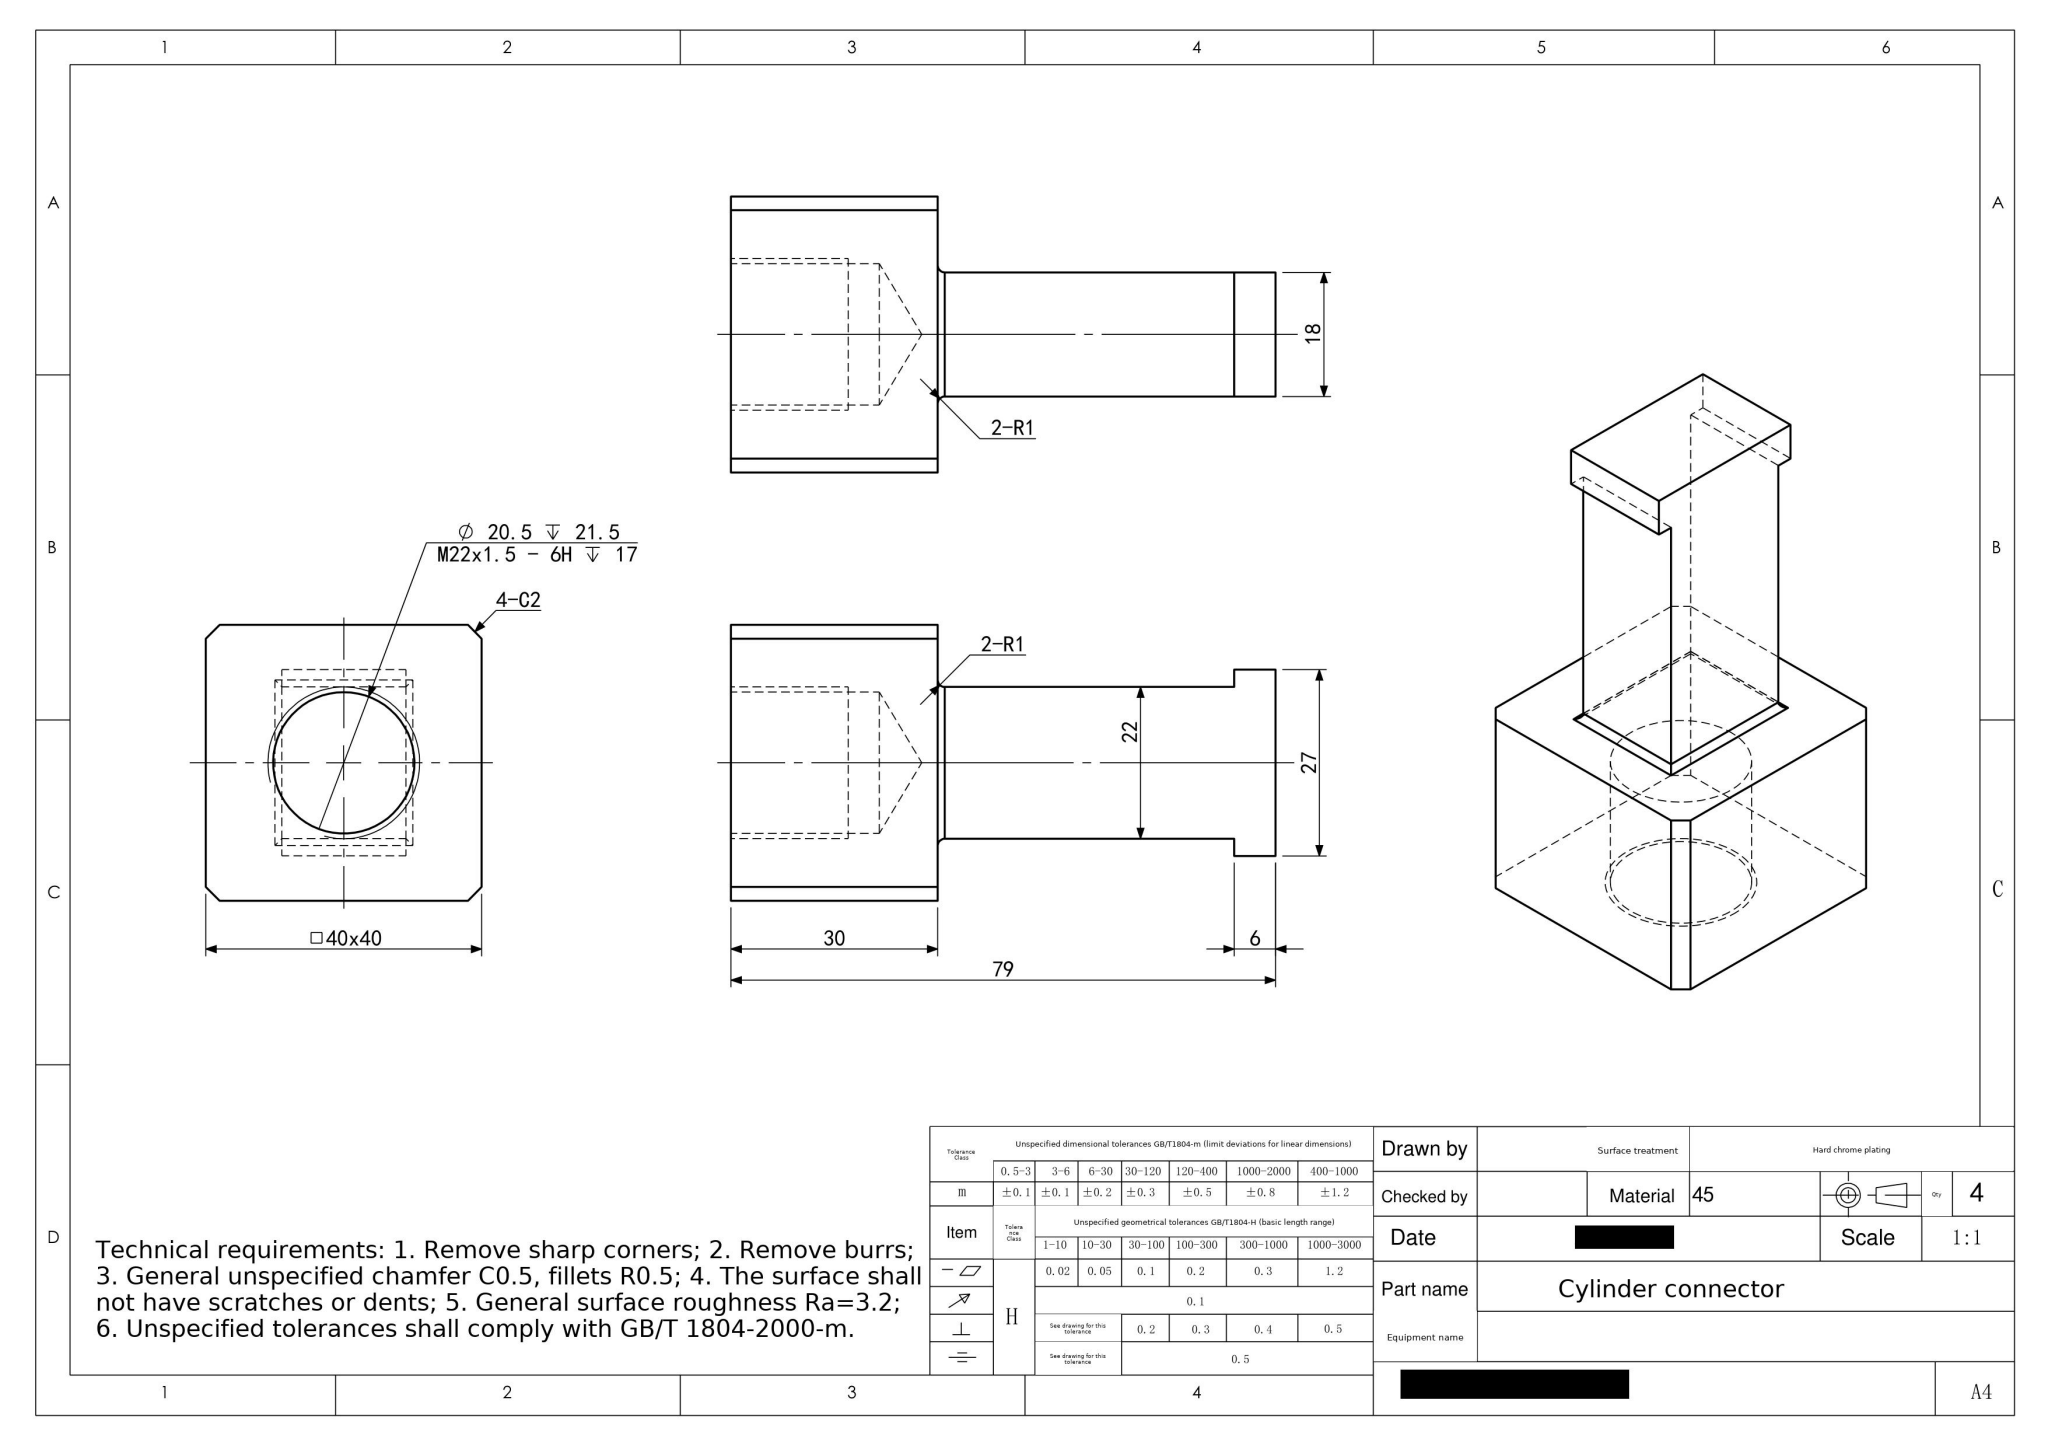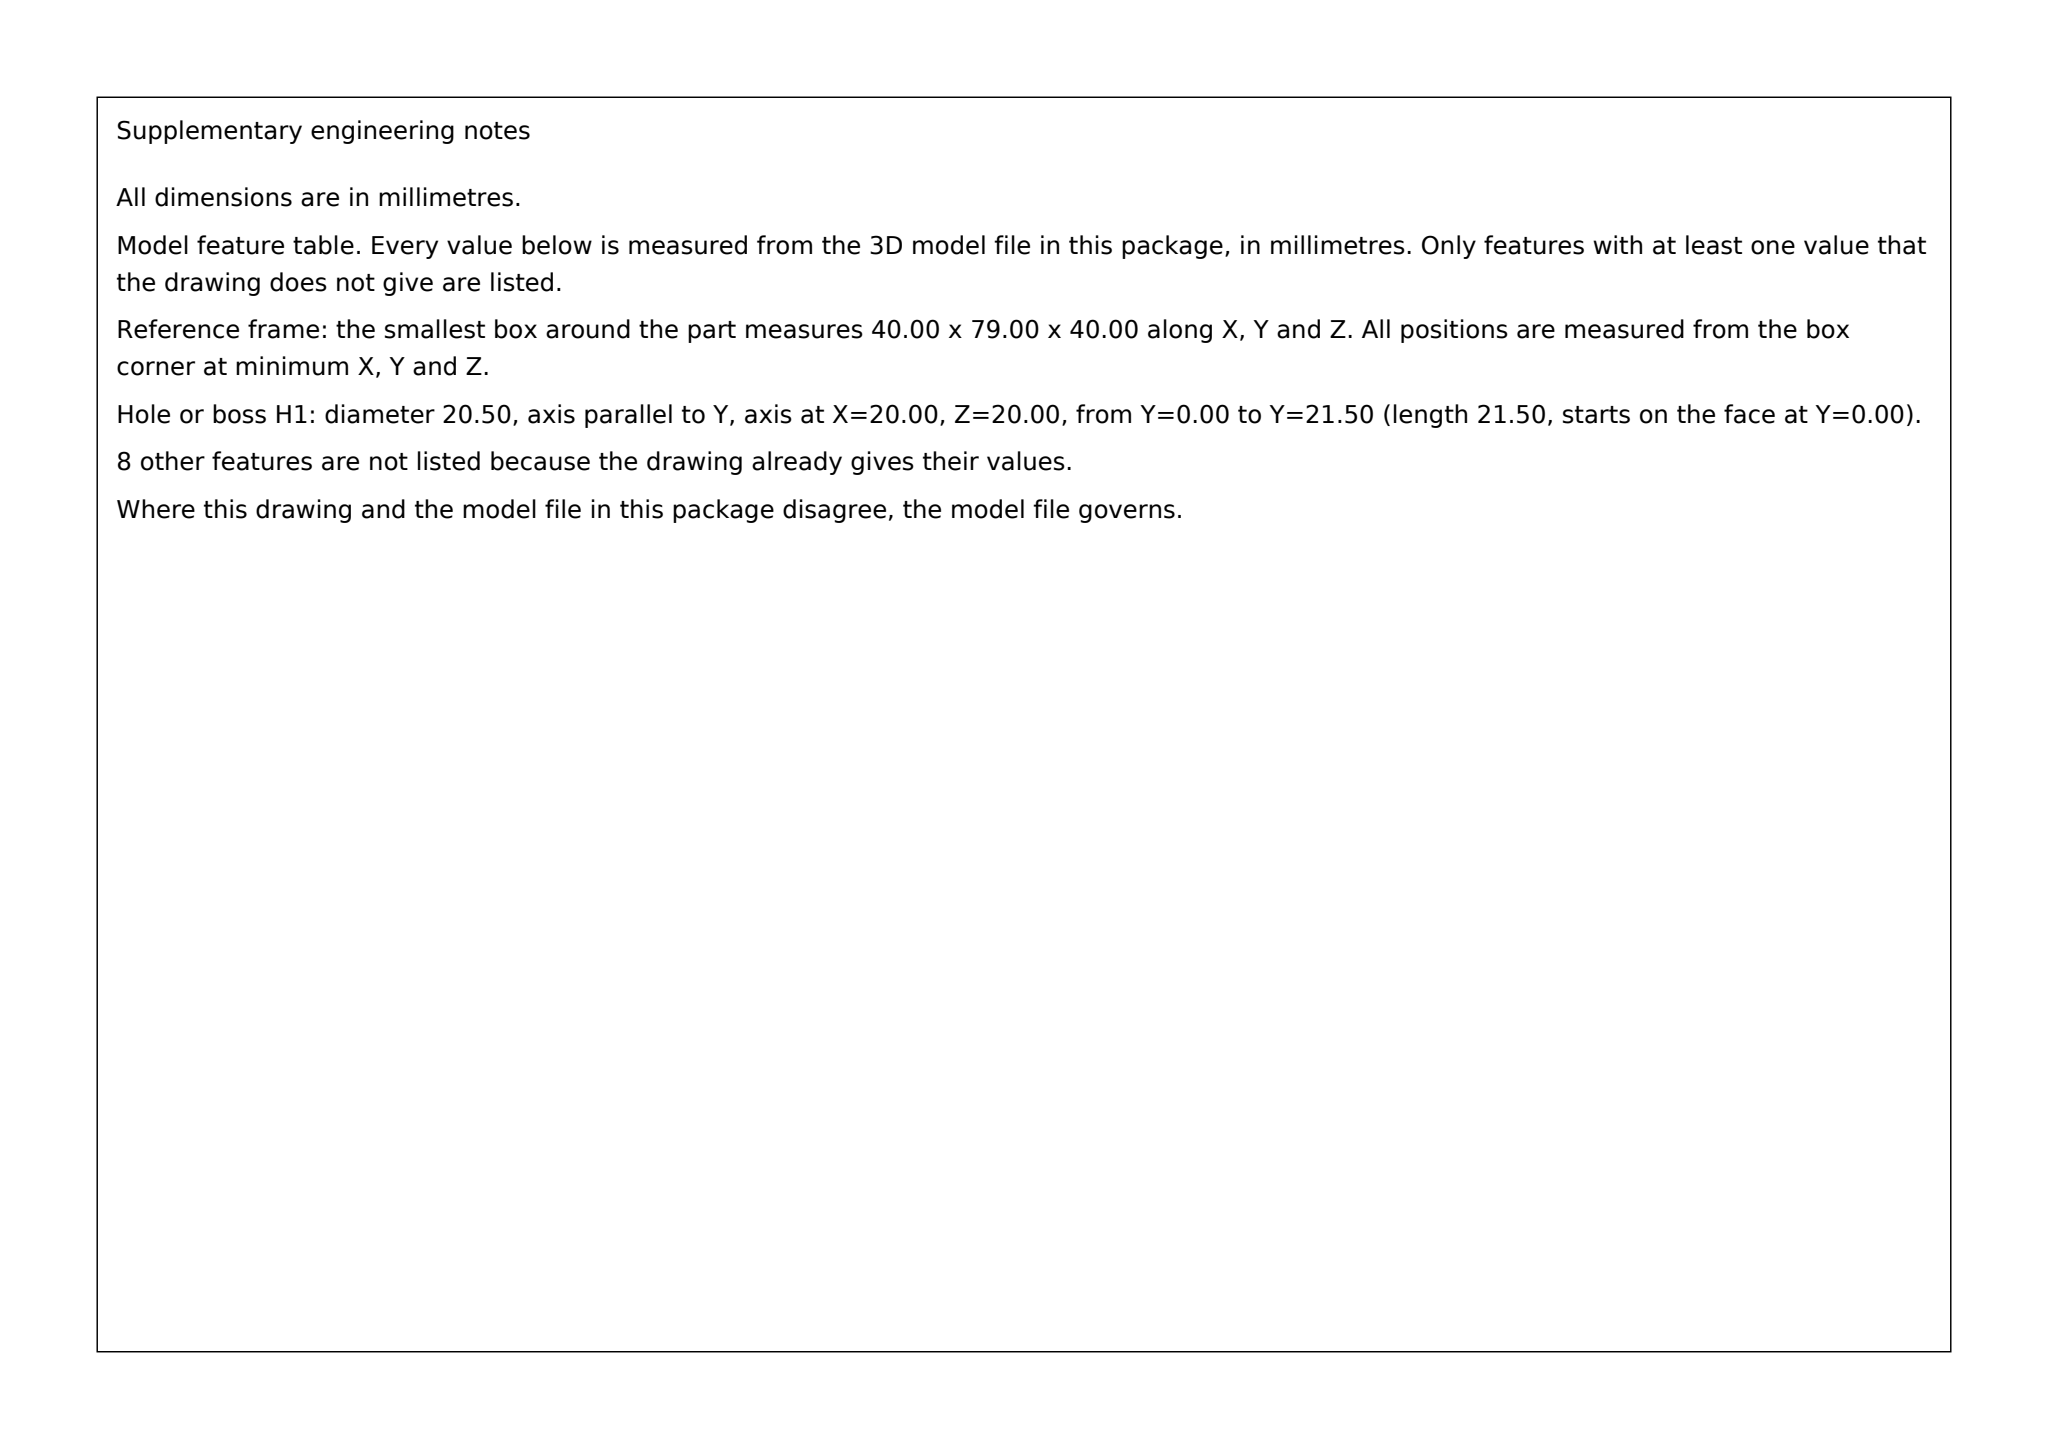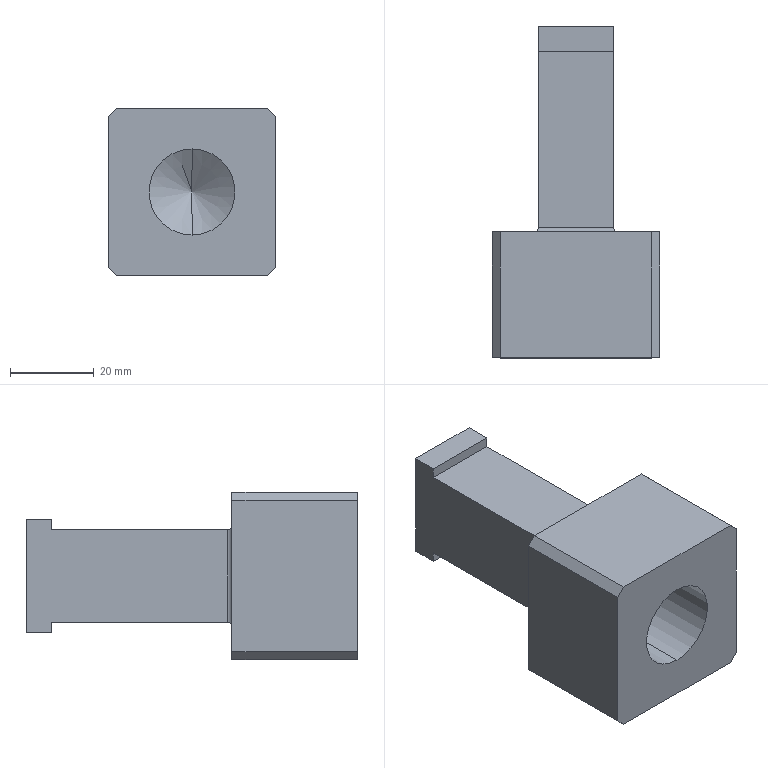Part | SolidWorks | mm | material 45 | 1 solid | 27 faces | box 40 x 79 x 40 mm | volume 59948 mm3 | plane 19 | cylinder 6 | cone 2 | commonest cylinder face diameters 2 x4 20.5 x2
build123d program:
from build123d import *

# Parameters (mm, degrees)
BOSS_EXTRUDE1_DEPTH        = 20
M22X1_5_TAPPED_HOLE1_D     = 20.5
M22X1_5_TAPPED_HOLE1_DEPTH = 21.5
M22X1_5_TAPPED_HOLE1_TIP   = 6.159
CUT_EXTRUDE1_REACH         = 85.911
SKETCH4_W                  = 11
SKETCH4_H                  = 27
FILLET1_R                  = 1
CHAMFER1_SIZE              = 2


with BuildPart() as part:
    # Sketch1 → Boss-Extrude1 (new, symmetric)
    with BuildSketch(Plane(origin=(0, 0, 0), x_dir=(0, 0, -1), z_dir=(1, 0, 0))):
        Polygon((13.5, 0), (13.5, -6), (11, -6), (11, -49), (20, -49), (20, -79), (-20, -79), (-20, -49), (-11, -49), (-11, -6), (-13.5, -6), (-13.5, 0), align=None)
    extrude(amount=BOSS_EXTRUDE1_DEPTH, both=True)

    # M22x1.5 Tapped Hole1
    with Locations(Plane(origin=(0, -79, 0), x_dir=(-1, 0, 0), z_dir=(0, -1, 0))):
        with Locations((0, 0)):
            Hole(M22X1_5_TAPPED_HOLE1_D / 2, depth=M22X1_5_TAPPED_HOLE1_DEPTH)
            with Locations((0, 0, -(M22X1_5_TAPPED_HOLE1_DEPTH + M22X1_5_TAPPED_HOLE1_TIP / 2))):  # 118° drill point
                Cone(0, M22X1_5_TAPPED_HOLE1_D / 2, M22X1_5_TAPPED_HOLE1_TIP, mode=Mode.SUBTRACT)

    # Cut-Extrude1: up to this face of the body (flat: up to its plane)
    cut_extrude1_end = Plane(part.part.faces().sort_by_distance((0, -49, -15.5))[0])
    # Sketch4 → Cut-Extrude1 (cut, up to the picked face)
    with BuildSketch(Plane(origin=(0, 0, 0), x_dir=(1, 0, 0), z_dir=(0, 1, 0)), mode=Mode.PRIVATE) as cut_extrude1_sk1:
        with Locations((-14.5, 0)):
            Rectangle(SKETCH4_W, SKETCH4_H)
    cut_extrude1_tool1 = split(extrude(cut_extrude1_sk1.sketch, amount=-CUT_EXTRUDE1_REACH, mode=Mode.PRIVATE), bisect_by=cut_extrude1_end, keep=Keep.BOTH, mode=Mode.PRIVATE)
    # Sketch4 → Cut-Extrude1 (cut, up to the picked face)
    with BuildSketch(Plane(origin=(0, 0, 0), x_dir=(1, 0, 0), z_dir=(0, 1, 0)), mode=Mode.PRIVATE) as cut_extrude1_sk2:
        with Locations((14.5, 0)):
            Rectangle(SKETCH4_W, SKETCH4_H)
    cut_extrude1_tool2 = split(extrude(cut_extrude1_sk2.sketch, amount=-CUT_EXTRUDE1_REACH, mode=Mode.PRIVATE), bisect_by=cut_extrude1_end, keep=Keep.BOTH, mode=Mode.PRIVATE)
    add(cut_extrude1_tool1.solids().sort_by(Axis((-14.5, 0, 0), (0, -1, 0)))[0], mode=Mode.SUBTRACT)
    add(cut_extrude1_tool2.solids().sort_by(Axis((14.5, 0, 0), (0, -1, 0)))[0], mode=Mode.SUBTRACT)

    # Fillet1
    fillet1_edges = [part.edges().sort_by_distance(p)[0] for p in [
        (0, -49, -11),
        (0, -49, 11),
        (-9, -49, 0),
        (9, -49, 0),
    ]]
    fillet(fillet1_edges, radius=FILLET1_R)

    # Chamfer1
    chamfer1_edges = [part.edges().sort_by_distance(p)[0] for p in [
        (-20, -64, -20),
        (-20, -64, 20),
        (20, -64, 20),
        (20, -64, -20),
    ]]
    chamfer(chamfer1_edges, length=CHAMFER1_SIZE)


solid = part.part
STEP:
#1=CARTESIAN_POINT('',(0.,-57.5,10.25));
#2=VERTEX_POINT('',#1);
#3=CARTESIAN_POINT('',(0.,-57.5,-10.25));
#4=VERTEX_POINT('',#3);
#5=CARTESIAN_POINT('',(0.,-57.5,0.));
#6=DIRECTION('',(0.,-1.,0.));
#7=DIRECTION('',(0.,0.,-1.));
#8=AXIS2_PLACEMENT_3D('',#5,#6,#7);
#9=CIRCLE('',#8,10.25);
#10=EDGE_CURVE('',#2,#4,#9,.T.);
#11=ORIENTED_EDGE('',*,*,#10,.F.);
#12=CARTESIAN_POINT('',(0.,-79.,10.25));
#13=VERTEX_POINT('',#12);
#14=CARTESIAN_POINT('',(0.,-79.,10.25));
#15=DIRECTION('',(0.,-1.,0.));
#16=VECTOR('',#15,1000.);
#17=LINE('',#14,#16);
#18=EDGE_CURVE('',#2,#13,#17,.T.);
#19=ORIENTED_EDGE('',*,*,#18,.T.);
#20=CARTESIAN_POINT('',(0.,-79.,-10.25));
#21=VERTEX_POINT('',#20);
#22=CARTESIAN_POINT('',(0.,-79.,0.));
#23=DIRECTION('',(0.,-1.,0.));
#24=DIRECTION('',(0.,0.,-1.));
#25=AXIS2_PLACEMENT_3D('',#22,#23,#24);
#26=CIRCLE('',#25,10.25);
#27=EDGE_CURVE('',#13,#21,#26,.T.);
#28=ORIENTED_EDGE('',*,*,#27,.T.);
#29=CARTESIAN_POINT('',(0.,-79.,-10.25));
#30=DIRECTION('',(0.,-1.,0.));
#31=VECTOR('',#30,1000.);
#32=LINE('',#29,#31);
#33=EDGE_CURVE('',#4,#21,#32,.T.);
#34=ORIENTED_EDGE('',*,*,#33,.F.);
#35=EDGE_LOOP('',(#11,#19,#28,#34));
#36=FACE_OUTER_BOUND('',#35,.T.);
#37=CARTESIAN_POINT('',(0.,-79.,0.));
#38=DIRECTION('',(0.,-1.,0.));
#39=DIRECTION('',(0.,0.,-1.));
#40=AXIS2_PLACEMENT_3D('',#37,#38,#39);
#41=CYLINDRICAL_SURFACE('',#40,10.25);
#42=ADVANCED_FACE('',(#36),#41,.F.);
#43=CARTESIAN_POINT('',(-0.,-51.341,0.));
#44=VERTEX_POINT('',#43);
#45=CARTESIAN_POINT('',(0.,-57.5,-10.25));
#46=DIRECTION('',(0.,-0.515,-0.8572));
#47=VECTOR('',#46,1000.);
#48=LINE('',#45,#47);
#49=EDGE_CURVE('',#44,#4,#48,.T.);
#50=ORIENTED_EDGE('',*,*,#49,.F.);
#51=CARTESIAN_POINT('',(0.,-57.5,10.25));
#52=DIRECTION('',(0.,-0.515,0.8572));
#53=VECTOR('',#52,1000.);
#54=LINE('',#51,#53);
#55=EDGE_CURVE('',#44,#2,#54,.T.);
#56=ORIENTED_EDGE('',*,*,#55,.T.);
#57=ORIENTED_EDGE('',*,*,#10,.T.);
#58=EDGE_LOOP('',(#50,#56,#57));
#59=FACE_OUTER_BOUND('',#58,.T.);
#60=CARTESIAN_POINT('',(0.,-57.5,0.));
#61=DIRECTION('',(0.,-1.,0.));
#62=DIRECTION('',(0.,0.,-1.));
#63=AXIS2_PLACEMENT_3D('',#60,#61,#62);
#64=CONICAL_SURFACE('',#63,10.25,1.03);
#65=ADVANCED_FACE('',(#59),#64,.F.);
#66=CARTESIAN_POINT('',(9.,-6.,-11.));
#67=VERTEX_POINT('',#66);
#68=CARTESIAN_POINT('',(-9.,-6.,-11.));
#69=VERTEX_POINT('',#68);
#70=CARTESIAN_POINT('',(20.,-6.,-11.));
#71=DIRECTION('',(-1.,0.,0.));
#72=VECTOR('',#71,1000.);
#73=LINE('',#70,#72);
#74=EDGE_CURVE('',#67,#69,#73,.T.);
#75=ORIENTED_EDGE('',*,*,#74,.T.);
#76=CARTESIAN_POINT('',(-9.,-6.,-13.5));
#77=VERTEX_POINT('',#76);
#78=CARTESIAN_POINT('',(-9.,-6.,-13.5));
#79=DIRECTION('',(-0.,0.,-1.));
#80=VECTOR('',#79,1000.);
#81=LINE('',#78,#80);
#82=EDGE_CURVE('',#69,#77,#81,.T.);
#83=ORIENTED_EDGE('',*,*,#82,.T.);
#84=CARTESIAN_POINT('',(9.,-6.,-13.5));
#85=VERTEX_POINT('',#84);
#86=CARTESIAN_POINT('',(20.,-6.,-13.5));
#87=DIRECTION('',(-1.,0.,0.));
#88=VECTOR('',#87,1000.);
#89=LINE('',#86,#88);
#90=EDGE_CURVE('',#85,#77,#89,.T.);
#91=ORIENTED_EDGE('',*,*,#90,.F.);
#92=CARTESIAN_POINT('',(9.,-6.,-13.5));
#93=DIRECTION('',(0.,-0.,1.));
#94=VECTOR('',#93,1000.);
#95=LINE('',#92,#94);
#96=EDGE_CURVE('',#85,#67,#95,.T.);
#97=ORIENTED_EDGE('',*,*,#96,.T.);
#98=EDGE_LOOP('',(#75,#83,#91,#97));
#99=FACE_OUTER_BOUND('',#98,.T.);
#100=CARTESIAN_POINT('',(20.,-6.,-13.5));
#101=DIRECTION('',(0.,1.,0.));
#102=DIRECTION('',(0.,-0.,1.));
#103=AXIS2_PLACEMENT_3D('',#100,#101,#102);
#104=PLANE('',#103);
#105=ADVANCED_FACE('',(#99),#104,.F.);
#106=ORIENTED_EDGE('',*,*,#90,.T.);
#107=CARTESIAN_POINT('',(-9.,0.,-13.5));
#108=VERTEX_POINT('',#107);
#109=CARTESIAN_POINT('',(-9.,-78.155,-13.5));
#110=DIRECTION('',(0.,1.,0.));
#111=VECTOR('',#110,1000.);
#112=LINE('',#109,#111);
#113=EDGE_CURVE('',#77,#108,#112,.T.);
#114=ORIENTED_EDGE('',*,*,#113,.T.);
#115=CARTESIAN_POINT('',(9.,0.,-13.5));
#116=VERTEX_POINT('',#115);
#117=CARTESIAN_POINT('',(20.,0.,-13.5));
#118=DIRECTION('',(-1.,0.,0.));
#119=VECTOR('',#118,1000.);
#120=LINE('',#117,#119);
#121=EDGE_CURVE('',#116,#108,#120,.T.);
#122=ORIENTED_EDGE('',*,*,#121,.F.);
#123=CARTESIAN_POINT('',(9.,-78.155,-13.5));
#124=DIRECTION('',(0.,1.,0.));
#125=VECTOR('',#124,1000.);
#126=LINE('',#123,#125);
#127=EDGE_CURVE('',#85,#116,#126,.T.);
#128=ORIENTED_EDGE('',*,*,#127,.F.);
#129=EDGE_LOOP('',(#106,#114,#122,#128));
#130=FACE_OUTER_BOUND('',#129,.T.);
#131=CARTESIAN_POINT('',(20.,0.,-13.5));
#132=DIRECTION('',(0.,0.,1.));
#133=DIRECTION('',(1.,0.,0.));
#134=AXIS2_PLACEMENT_3D('',#131,#132,#133);
#135=PLANE('',#134);
#136=ADVANCED_FACE('',(#130),#135,.F.);
#137=ORIENTED_EDGE('',*,*,#121,.T.);
#138=CARTESIAN_POINT('',(-9.,-0.,13.5));
#139=VERTEX_POINT('',#138);
#140=CARTESIAN_POINT('',(-9.,0.,-13.5));
#141=DIRECTION('',(-0.,0.,-1.));
#142=VECTOR('',#141,1000.);
#143=LINE('',#140,#142);
#144=EDGE_CURVE('',#139,#108,#143,.T.);
#145=ORIENTED_EDGE('',*,*,#144,.F.);
#146=CARTESIAN_POINT('',(9.,-0.,13.5));
#147=VERTEX_POINT('',#146);
#148=CARTESIAN_POINT('',(20.,-0.,13.5));
#149=DIRECTION('',(-1.,0.,0.));
#150=VECTOR('',#149,1000.);
#151=LINE('',#148,#150);
#152=EDGE_CURVE('',#147,#139,#151,.T.);
#153=ORIENTED_EDGE('',*,*,#152,.F.);
#154=CARTESIAN_POINT('',(9.,0.,-13.5));
#155=DIRECTION('',(0.,-0.,1.));
#156=VECTOR('',#155,1000.);
#157=LINE('',#154,#156);
#158=EDGE_CURVE('',#116,#147,#157,.T.);
#159=ORIENTED_EDGE('',*,*,#158,.F.);
#160=EDGE_LOOP('',(#137,#145,#153,#159));
#161=FACE_OUTER_BOUND('',#160,.T.);
#162=CARTESIAN_POINT('',(20.,0.,-13.5));
#163=DIRECTION('',(0.,-1.,-0.));
#164=DIRECTION('',(0.,0.,-1.));
#165=AXIS2_PLACEMENT_3D('',#162,#163,#164);
#166=PLANE('',#165);
#167=ADVANCED_FACE('',(#161),#166,.F.);
#168=ORIENTED_EDGE('',*,*,#152,.T.);
#169=CARTESIAN_POINT('',(-9.,-6.,13.5));
#170=VERTEX_POINT('',#169);
#171=CARTESIAN_POINT('',(-9.,-78.155,13.5));
#172=DIRECTION('',(0.,1.,0.));
#173=VECTOR('',#172,1000.);
#174=LINE('',#171,#173);
#175=EDGE_CURVE('',#170,#139,#174,.T.);
#176=ORIENTED_EDGE('',*,*,#175,.F.);
#177=CARTESIAN_POINT('',(9.,-6.,13.5));
#178=VERTEX_POINT('',#177);
#179=CARTESIAN_POINT('',(20.,-6.,13.5));
#180=DIRECTION('',(-1.,0.,0.));
#181=VECTOR('',#180,1000.);
#182=LINE('',#179,#181);
#183=EDGE_CURVE('',#178,#170,#182,.T.);
#184=ORIENTED_EDGE('',*,*,#183,.F.);
#185=CARTESIAN_POINT('',(9.,-78.155,13.5));
#186=DIRECTION('',(0.,1.,0.));
#187=VECTOR('',#186,1000.);
#188=LINE('',#185,#187);
#189=EDGE_CURVE('',#178,#147,#188,.T.);
#190=ORIENTED_EDGE('',*,*,#189,.T.);
#191=EDGE_LOOP('',(#168,#176,#184,#190));
#192=FACE_OUTER_BOUND('',#191,.T.);
#193=CARTESIAN_POINT('',(20.,-0.,13.5));
#194=DIRECTION('',(0.,0.,-1.));
#195=DIRECTION('',(-1.,0.,0.));
#196=AXIS2_PLACEMENT_3D('',#193,#194,#195);
#197=PLANE('',#196);
#198=ADVANCED_FACE('',(#192),#197,.F.);
#199=ORIENTED_EDGE('',*,*,#183,.T.);
#200=CARTESIAN_POINT('',(-9.,-6.,11.));
#201=VERTEX_POINT('',#200);
#202=CARTESIAN_POINT('',(-9.,-6.,13.5));
#203=DIRECTION('',(-0.,0.,-1.));
#204=VECTOR('',#203,1000.);
#205=LINE('',#202,#204);
#206=EDGE_CURVE('',#170,#201,#205,.T.);
#207=ORIENTED_EDGE('',*,*,#206,.T.);
#208=CARTESIAN_POINT('',(9.,-6.,11.));
#209=VERTEX_POINT('',#208);
#210=CARTESIAN_POINT('',(20.,-6.,11.));
#211=DIRECTION('',(-1.,0.,0.));
#212=VECTOR('',#211,1000.);
#213=LINE('',#210,#212);
#214=EDGE_CURVE('',#209,#201,#213,.T.);
#215=ORIENTED_EDGE('',*,*,#214,.F.);
#216=CARTESIAN_POINT('',(9.,-6.,13.5));
#217=DIRECTION('',(0.,0.,1.));
#218=VECTOR('',#217,1000.);
#219=LINE('',#216,#218);
#220=EDGE_CURVE('',#209,#178,#219,.T.);
#221=ORIENTED_EDGE('',*,*,#220,.T.);
#222=EDGE_LOOP('',(#199,#207,#215,#221));
#223=FACE_OUTER_BOUND('',#222,.T.);
#224=CARTESIAN_POINT('',(20.,-6.,13.5));
#225=DIRECTION('',(0.,1.,0.));
#226=DIRECTION('',(0.,0.,1.));
#227=AXIS2_PLACEMENT_3D('',#224,#225,#226);
#228=PLANE('',#227);
#229=ADVANCED_FACE('',(#223),#228,.F.);
#230=CARTESIAN_POINT('',(-9.,-48.,11.));
#231=VERTEX_POINT('',#230);
#232=CARTESIAN_POINT('',(-9.,-6.,11.));
#233=DIRECTION('',(-0.,-1.,-0.));
#234=VECTOR('',#233,1000.);
#235=LINE('',#232,#234);
#236=EDGE_CURVE('',#201,#231,#235,.T.);
#237=ORIENTED_EDGE('',*,*,#236,.T.);
#238=CARTESIAN_POINT('',(9.,-48.,11.));
#239=VERTEX_POINT('',#238);
#240=CARTESIAN_POINT('',(9.,-48.,11.));
#241=DIRECTION('',(1.,0.,0.));
#242=VECTOR('',#241,1000.);
#243=LINE('',#240,#242);
#244=EDGE_CURVE('',#231,#239,#243,.T.);
#245=ORIENTED_EDGE('',*,*,#244,.T.);
#246=CARTESIAN_POINT('',(9.,-6.,11.));
#247=DIRECTION('',(0.,1.,0.));
#248=VECTOR('',#247,1000.);
#249=LINE('',#246,#248);
#250=EDGE_CURVE('',#239,#209,#249,.T.);
#251=ORIENTED_EDGE('',*,*,#250,.T.);
#252=ORIENTED_EDGE('',*,*,#214,.T.);
#253=EDGE_LOOP('',(#237,#245,#251,#252));
#254=FACE_OUTER_BOUND('',#253,.T.);
#255=CARTESIAN_POINT('',(20.,-6.,11.));
#256=DIRECTION('',(0.,0.,-1.));
#257=DIRECTION('',(0.,1.,0.));
#258=AXIS2_PLACEMENT_3D('',#255,#256,#257);
#259=PLANE('',#258);
#260=ADVANCED_FACE('',(#254),#259,.F.);
#261=CARTESIAN_POINT('',(18.,-49.,20.));
#262=VERTEX_POINT('',#261);
#263=CARTESIAN_POINT('',(-18.,-49.,20.));
#264=VERTEX_POINT('',#263);
#265=CARTESIAN_POINT('',(20.,-49.,20.));
#266=DIRECTION('',(-1.,0.,0.));
#267=VECTOR('',#266,1000.);
#268=LINE('',#265,#267);
#269=EDGE_CURVE('',#262,#264,#268,.T.);
#270=ORIENTED_EDGE('',*,*,#269,.T.);
#271=CARTESIAN_POINT('',(-18.,-79.,20.));
#272=VERTEX_POINT('',#271);
#273=CARTESIAN_POINT('',(-18.,-49.,20.));
#274=DIRECTION('',(0.,-1.,0.));
#275=VECTOR('',#274,1000.);
#276=LINE('',#273,#275);
#277=EDGE_CURVE('',#264,#272,#276,.T.);
#278=ORIENTED_EDGE('',*,*,#277,.T.);
#279=CARTESIAN_POINT('',(18.,-79.,20.));
#280=VERTEX_POINT('',#279);
#281=CARTESIAN_POINT('',(20.,-79.,20.));
#282=DIRECTION('',(-1.,0.,0.));
#283=VECTOR('',#282,1000.);
#284=LINE('',#281,#283);
#285=EDGE_CURVE('',#280,#272,#284,.T.);
#286=ORIENTED_EDGE('',*,*,#285,.F.);
#287=CARTESIAN_POINT('',(18.,-49.,20.));
#288=DIRECTION('',(0.,1.,0.));
#289=VECTOR('',#288,1000.);
#290=LINE('',#287,#289);
#291=EDGE_CURVE('',#280,#262,#290,.T.);
#292=ORIENTED_EDGE('',*,*,#291,.T.);
#293=EDGE_LOOP('',(#270,#278,#286,#292));
#294=FACE_OUTER_BOUND('',#293,.T.);
#295=CARTESIAN_POINT('',(20.,-49.,20.));
#296=DIRECTION('',(0.,0.,-1.));
#297=DIRECTION('',(-1.,0.,0.));
#298=AXIS2_PLACEMENT_3D('',#295,#296,#297);
#299=PLANE('',#298);
#300=ADVANCED_FACE('',(#294),#299,.F.);
#301=CARTESIAN_POINT('',(0.,-79.,0.));
#302=DIRECTION('',(0.,-1.,0.));
#303=DIRECTION('',(0.,0.,-1.));
#304=AXIS2_PLACEMENT_3D('',#301,#302,#303);
#305=CIRCLE('',#304,10.25);
#306=EDGE_CURVE('',#21,#13,#305,.T.);
#307=ORIENTED_EDGE('',*,*,#306,.F.);
#308=ORIENTED_EDGE('',*,*,#27,.F.);
#309=EDGE_LOOP('',(#307,#308));
#310=FACE_BOUND('',#309,.T.);
#311=ORIENTED_EDGE('',*,*,#285,.T.);
#312=CARTESIAN_POINT('',(-20.,-79.,18.));
#313=VERTEX_POINT('',#312);
#314=CARTESIAN_POINT('',(-18.,-79.,20.));
#315=DIRECTION('',(-0.7071,0.,-0.7071));
#316=VECTOR('',#315,1000.);
#317=LINE('',#314,#316);
#318=EDGE_CURVE('',#272,#313,#317,.T.);
#319=ORIENTED_EDGE('',*,*,#318,.T.);
#320=CARTESIAN_POINT('',(-20.,-79.,-18.));
#321=VERTEX_POINT('',#320);
#322=CARTESIAN_POINT('',(-20.,-79.,20.));
#323=DIRECTION('',(0.,0.,-1.));
#324=VECTOR('',#323,1000.);
#325=LINE('',#322,#324);
#326=EDGE_CURVE('',#313,#321,#325,.T.);
#327=ORIENTED_EDGE('',*,*,#326,.T.);
#328=CARTESIAN_POINT('',(-18.,-79.,-20.));
#329=VERTEX_POINT('',#328);
#330=CARTESIAN_POINT('',(-18.,-79.,-20.));
#331=DIRECTION('',(0.7071,0.,-0.7071));
#332=VECTOR('',#331,1000.);
#333=LINE('',#330,#332);
#334=EDGE_CURVE('',#321,#329,#333,.T.);
#335=ORIENTED_EDGE('',*,*,#334,.T.);
#336=CARTESIAN_POINT('',(18.,-79.,-20.));
#337=VERTEX_POINT('',#336);
#338=CARTESIAN_POINT('',(20.,-79.,-20.));
#339=DIRECTION('',(-1.,0.,0.));
#340=VECTOR('',#339,1000.);
#341=LINE('',#338,#340);
#342=EDGE_CURVE('',#337,#329,#341,.T.);
#343=ORIENTED_EDGE('',*,*,#342,.F.);
#344=CARTESIAN_POINT('',(20.,-79.,-18.));
#345=VERTEX_POINT('',#344);
#346=CARTESIAN_POINT('',(20.,-79.,-18.));
#347=DIRECTION('',(0.7071,0.,0.7071));
#348=VECTOR('',#347,1000.);
#349=LINE('',#346,#348);
#350=EDGE_CURVE('',#337,#345,#349,.T.);
#351=ORIENTED_EDGE('',*,*,#350,.T.);
#352=CARTESIAN_POINT('',(20.,-79.,18.));
#353=VERTEX_POINT('',#352);
#354=CARTESIAN_POINT('',(20.,-79.,20.));
#355=DIRECTION('',(0.,0.,-1.));
#356=VECTOR('',#355,1000.);
#357=LINE('',#354,#356);
#358=EDGE_CURVE('',#353,#345,#357,.T.);
#359=ORIENTED_EDGE('',*,*,#358,.F.);
#360=CARTESIAN_POINT('',(20.,-79.,18.));
#361=DIRECTION('',(-0.7071,0.,0.7071));
#362=VECTOR('',#361,1000.);
#363=LINE('',#360,#362);
#364=EDGE_CURVE('',#353,#280,#363,.T.);
#365=ORIENTED_EDGE('',*,*,#364,.T.);
#366=EDGE_LOOP('',(#311,#319,#327,#335,#343,#351,#359,#365));
#367=FACE_OUTER_BOUND('',#366,.T.);
#368=CARTESIAN_POINT('',(20.,-79.,20.));
#369=DIRECTION('',(0.,1.,0.));
#370=DIRECTION('',(0.,0.,1.));
#371=AXIS2_PLACEMENT_3D('',#368,#369,#370);
#372=PLANE('',#371);
#373=ADVANCED_FACE('',(#310,#367),#372,.F.);
#374=CARTESIAN_POINT('',(18.,-49.,-20.));
#375=VERTEX_POINT('',#374);
#376=CARTESIAN_POINT('',(-18.,-49.,-20.));
#377=VERTEX_POINT('',#376);
#378=CARTESIAN_POINT('',(20.,-49.,-20.));
#379=DIRECTION('',(-1.,0.,0.));
#380=VECTOR('',#379,1000.);
#381=LINE('',#378,#380);
#382=EDGE_CURVE('',#375,#377,#381,.T.);
#383=ORIENTED_EDGE('',*,*,#382,.F.);
#384=CARTESIAN_POINT('',(18.,-79.,-20.));
#385=DIRECTION('',(0.,-1.,-0.));
#386=VECTOR('',#385,1000.);
#387=LINE('',#384,#386);
#388=EDGE_CURVE('',#375,#337,#387,.T.);
#389=ORIENTED_EDGE('',*,*,#388,.T.);
#390=ORIENTED_EDGE('',*,*,#342,.T.);
#391=CARTESIAN_POINT('',(-18.,-49.,-20.));
#392=DIRECTION('',(0.,1.,0.));
#393=VECTOR('',#392,1000.);
#394=LINE('',#391,#393);
#395=EDGE_CURVE('',#329,#377,#394,.T.);
#396=ORIENTED_EDGE('',*,*,#395,.T.);
#397=EDGE_LOOP('',(#383,#389,#390,#396));
#398=FACE_OUTER_BOUND('',#397,.T.);
#399=CARTESIAN_POINT('',(20.,-49.,-20.));
#400=DIRECTION('',(0.,-0.,1.));
#401=DIRECTION('',(0.,-1.,-0.));
#402=AXIS2_PLACEMENT_3D('',#399,#400,#401);
#403=PLANE('',#402);
#404=ADVANCED_FACE('',(#398),#403,.F.);
#405=CARTESIAN_POINT('',(10.,-49.,-12.));
#406=VERTEX_POINT('',#405);
#407=CARTESIAN_POINT('',(10.,-49.,12.));
#408=VERTEX_POINT('',#407);
#409=CARTESIAN_POINT('',(10.,-49.,11.));
#410=DIRECTION('',(0.,0.,1.));
#411=VECTOR('',#410,1000.);
#412=LINE('',#409,#411);
#413=EDGE_CURVE('',#406,#408,#412,.T.);
#414=ORIENTED_EDGE('',*,*,#413,.T.);
#415=CARTESIAN_POINT('',(-10.,-49.,12.));
#416=VERTEX_POINT('',#415);
#417=CARTESIAN_POINT('',(-9.,-49.,12.));
#418=DIRECTION('',(-1.,0.,0.));
#419=VECTOR('',#418,1000.);
#420=LINE('',#417,#419);
#421=EDGE_CURVE('',#408,#416,#420,.T.);
#422=ORIENTED_EDGE('',*,*,#421,.T.);
#423=CARTESIAN_POINT('',(-10.,-49.,-12.));
#424=VERTEX_POINT('',#423);
#425=CARTESIAN_POINT('',(-10.,-49.,-11.));
#426=DIRECTION('',(-0.,0.,-1.));
#427=VECTOR('',#426,1000.);
#428=LINE('',#425,#427);
#429=EDGE_CURVE('',#416,#424,#428,.T.);
#430=ORIENTED_EDGE('',*,*,#429,.T.);
#431=CARTESIAN_POINT('',(9.,-49.,-12.));
#432=DIRECTION('',(1.,0.,0.));
#433=VECTOR('',#432,1000.);
#434=LINE('',#431,#433);
#435=EDGE_CURVE('',#424,#406,#434,.T.);
#436=ORIENTED_EDGE('',*,*,#435,.T.);
#437=EDGE_LOOP('',(#414,#422,#430,#436));
#438=FACE_BOUND('',#437,.T.);
#439=CARTESIAN_POINT('',(-20.,-49.,-18.));
#440=VERTEX_POINT('',#439);
#441=CARTESIAN_POINT('',(-20.,-49.,18.));
#442=VERTEX_POINT('',#441);
#443=CARTESIAN_POINT('',(-20.,-49.,-11.));
#444=DIRECTION('',(0.,0.,1.));
#445=VECTOR('',#444,1000.);
#446=LINE('',#443,#445);
#447=EDGE_CURVE('',#440,#442,#446,.T.);
#448=ORIENTED_EDGE('',*,*,#447,.T.);
#449=CARTESIAN_POINT('',(-18.,-49.,20.));
#450=DIRECTION('',(0.7071,0.,0.7071));
#451=VECTOR('',#450,1000.);
#452=LINE('',#449,#451);
#453=EDGE_CURVE('',#442,#264,#452,.T.);
#454=ORIENTED_EDGE('',*,*,#453,.T.);
#455=ORIENTED_EDGE('',*,*,#269,.F.);
#456=CARTESIAN_POINT('',(20.,-49.,18.));
#457=VERTEX_POINT('',#456);
#458=CARTESIAN_POINT('',(20.,-49.,18.));
#459=DIRECTION('',(0.7071,0.,-0.7071));
#460=VECTOR('',#459,1000.);
#461=LINE('',#458,#460);
#462=EDGE_CURVE('',#262,#457,#461,.T.);
#463=ORIENTED_EDGE('',*,*,#462,.T.);
#464=CARTESIAN_POINT('',(20.,-49.,-18.));
#465=VERTEX_POINT('',#464);
#466=CARTESIAN_POINT('',(20.,-49.,11.));
#467=DIRECTION('',(0.,-0.,1.));
#468=VECTOR('',#467,1000.);
#469=LINE('',#466,#468);
#470=EDGE_CURVE('',#465,#457,#469,.T.);
#471=ORIENTED_EDGE('',*,*,#470,.F.);
#472=CARTESIAN_POINT('',(20.,-49.,-18.));
#473=DIRECTION('',(-0.7071,0.,-0.7071));
#474=VECTOR('',#473,1000.);
#475=LINE('',#472,#474);
#476=EDGE_CURVE('',#465,#375,#475,.T.);
#477=ORIENTED_EDGE('',*,*,#476,.T.);
#478=ORIENTED_EDGE('',*,*,#382,.T.);
#479=CARTESIAN_POINT('',(-18.,-49.,-20.));
#480=DIRECTION('',(-0.7071,0.,0.7071));
#481=VECTOR('',#480,1000.);
#482=LINE('',#479,#481);
#483=EDGE_CURVE('',#377,#440,#482,.T.);
#484=ORIENTED_EDGE('',*,*,#483,.T.);
#485=EDGE_LOOP('',(#448,#454,#455,#463,#471,#477,#478,#484));
#486=FACE_OUTER_BOUND('',#485,.T.);
#487=CARTESIAN_POINT('',(20.,-49.,-11.));
#488=DIRECTION('',(0.,-1.,0.));
#489=DIRECTION('',(0.,0.,-1.));
#490=AXIS2_PLACEMENT_3D('',#487,#488,#489);
#491=PLANE('',#490);
#492=ADVANCED_FACE('',(#438,#486),#491,.F.);
#493=CARTESIAN_POINT('',(9.,-48.,-11.));
#494=VERTEX_POINT('',#493);
#495=CARTESIAN_POINT('',(9.,-6.,-11.));
#496=DIRECTION('',(0.,-1.,-0.));
#497=VECTOR('',#496,1000.);
#498=LINE('',#495,#497);
#499=EDGE_CURVE('',#67,#494,#498,.T.);
#500=ORIENTED_EDGE('',*,*,#499,.T.);
#501=CARTESIAN_POINT('',(-9.,-48.,-11.));
#502=VERTEX_POINT('',#501);
#503=CARTESIAN_POINT('',(-9.,-48.,-11.));
#504=DIRECTION('',(-1.,0.,0.));
#505=VECTOR('',#504,1000.);
#506=LINE('',#503,#505);
#507=EDGE_CURVE('',#494,#502,#506,.T.);
#508=ORIENTED_EDGE('',*,*,#507,.T.);
#509=CARTESIAN_POINT('',(-9.,-6.,-11.));
#510=DIRECTION('',(-0.,1.,0.));
#511=VECTOR('',#510,1000.);
#512=LINE('',#509,#511);
#513=EDGE_CURVE('',#502,#69,#512,.T.);
#514=ORIENTED_EDGE('',*,*,#513,.T.);
#515=ORIENTED_EDGE('',*,*,#74,.F.);
#516=EDGE_LOOP('',(#500,#508,#514,#515));
#517=FACE_OUTER_BOUND('',#516,.T.);
#518=CARTESIAN_POINT('',(20.,-6.,-11.));
#519=DIRECTION('',(0.,-0.,1.));
#520=DIRECTION('',(0.,-1.,-0.));
#521=AXIS2_PLACEMENT_3D('',#518,#519,#520);
#522=PLANE('',#521);
#523=ADVANCED_FACE('',(#517),#522,.F.);
#524=ORIENTED_EDGE('',*,*,#470,.T.);
#525=CARTESIAN_POINT('',(20.,-79.,18.));
#526=DIRECTION('',(0.,-1.,0.));
#527=VECTOR('',#526,1000.);
#528=LINE('',#525,#527);
#529=EDGE_CURVE('',#457,#353,#528,.T.);
#530=ORIENTED_EDGE('',*,*,#529,.T.);
#531=ORIENTED_EDGE('',*,*,#358,.T.);
#532=CARTESIAN_POINT('',(20.,-49.,-18.));
#533=DIRECTION('',(0.,1.,0.));
#534=VECTOR('',#533,1000.);
#535=LINE('',#532,#534);
#536=EDGE_CURVE('',#345,#465,#535,.T.);
#537=ORIENTED_EDGE('',*,*,#536,.T.);
#538=EDGE_LOOP('',(#524,#530,#531,#537));
#539=FACE_OUTER_BOUND('',#538,.T.);
#540=CARTESIAN_POINT('',(20.,0.,0.));
#541=DIRECTION('',(1.,0.,0.));
#542=DIRECTION('',(0.,0.,-1.));
#543=AXIS2_PLACEMENT_3D('',#540,#541,#542);
#544=PLANE('',#543);
#545=ADVANCED_FACE('',(#539),#544,.T.);
#546=ORIENTED_EDGE('',*,*,#326,.F.);
#547=CARTESIAN_POINT('',(-20.,0.,18.));
#548=DIRECTION('',(0.,1.,0.));
#549=VECTOR('',#548,1000.);
#550=LINE('',#547,#549);
#551=EDGE_CURVE('',#313,#442,#550,.T.);
#552=ORIENTED_EDGE('',*,*,#551,.T.);
#553=ORIENTED_EDGE('',*,*,#447,.F.);
#554=CARTESIAN_POINT('',(-20.,0.,-18.));
#555=DIRECTION('',(0.,-1.,-0.));
#556=VECTOR('',#555,1000.);
#557=LINE('',#554,#556);
#558=EDGE_CURVE('',#440,#321,#557,.T.);
#559=ORIENTED_EDGE('',*,*,#558,.T.);
#560=EDGE_LOOP('',(#546,#552,#553,#559));
#561=FACE_OUTER_BOUND('',#560,.T.);
#562=CARTESIAN_POINT('',(-20.,0.,0.));
#563=DIRECTION('',(1.,0.,0.));
#564=DIRECTION('',(0.,0.,-1.));
#565=AXIS2_PLACEMENT_3D('',#562,#563,#564);
#566=PLANE('',#565);
#567=ADVANCED_FACE('',(#561),#566,.F.);
#568=ORIENTED_EDGE('',*,*,#55,.F.);
#569=ORIENTED_EDGE('',*,*,#49,.T.);
#570=CARTESIAN_POINT('',(0.,-57.5,0.));
#571=DIRECTION('',(0.,-1.,0.));
#572=DIRECTION('',(0.,0.,-1.));
#573=AXIS2_PLACEMENT_3D('',#570,#571,#572);
#574=CIRCLE('',#573,10.25);
#575=EDGE_CURVE('',#4,#2,#574,.T.);
#576=ORIENTED_EDGE('',*,*,#575,.T.);
#577=EDGE_LOOP('',(#568,#569,#576));
#578=FACE_OUTER_BOUND('',#577,.T.);
#579=CARTESIAN_POINT('',(0.,-57.5,0.));
#580=DIRECTION('',(0.,-1.,0.));
#581=DIRECTION('',(0.,0.,-1.));
#582=AXIS2_PLACEMENT_3D('',#579,#580,#581);
#583=CONICAL_SURFACE('',#582,10.25,1.03);
#584=ADVANCED_FACE('',(#578),#583,.F.);
#585=ORIENTED_EDGE('',*,*,#18,.F.);
#586=ORIENTED_EDGE('',*,*,#575,.F.);
#587=ORIENTED_EDGE('',*,*,#33,.T.);
#588=ORIENTED_EDGE('',*,*,#306,.T.);
#589=EDGE_LOOP('',(#585,#586,#587,#588));
#590=FACE_OUTER_BOUND('',#589,.T.);
#591=CARTESIAN_POINT('',(0.,-79.,0.));
#592=DIRECTION('',(0.,-1.,0.));
#593=DIRECTION('',(0.,0.,-1.));
#594=AXIS2_PLACEMENT_3D('',#591,#592,#593);
#595=CYLINDRICAL_SURFACE('',#594,10.25);
#596=ADVANCED_FACE('',(#590),#595,.F.);
#597=ORIENTED_EDGE('',*,*,#513,.F.);
#598=CARTESIAN_POINT('',(-9.,-48.,11.));
#599=DIRECTION('',(0.,0.,1.));
#600=VECTOR('',#599,1000.);
#601=LINE('',#598,#600);
#602=EDGE_CURVE('',#502,#231,#601,.T.);
#603=ORIENTED_EDGE('',*,*,#602,.T.);
#604=ORIENTED_EDGE('',*,*,#236,.F.);
#605=ORIENTED_EDGE('',*,*,#206,.F.);
#606=ORIENTED_EDGE('',*,*,#175,.T.);
#607=ORIENTED_EDGE('',*,*,#144,.T.);
#608=ORIENTED_EDGE('',*,*,#113,.F.);
#609=ORIENTED_EDGE('',*,*,#82,.F.);
#610=EDGE_LOOP('',(#597,#603,#604,#605,#606,#607,#608,#609));
#611=FACE_OUTER_BOUND('',#610,.T.);
#612=CARTESIAN_POINT('',(-9.,-78.155,-13.5));
#613=DIRECTION('',(1.,0.,-0.));
#614=DIRECTION('',(-0.,0.,-1.));
#615=AXIS2_PLACEMENT_3D('',#612,#613,#614);
#616=PLANE('',#615);
#617=ADVANCED_FACE('',(#611),#616,.F.);
#618=ORIENTED_EDGE('',*,*,#250,.F.);
#619=CARTESIAN_POINT('',(9.,-48.,-11.));
#620=DIRECTION('',(-0.,0.,-1.));
#621=VECTOR('',#620,1000.);
#622=LINE('',#619,#621);
#623=EDGE_CURVE('',#239,#494,#622,.T.);
#624=ORIENTED_EDGE('',*,*,#623,.T.);
#625=ORIENTED_EDGE('',*,*,#499,.F.);
#626=ORIENTED_EDGE('',*,*,#96,.F.);
#627=ORIENTED_EDGE('',*,*,#127,.T.);
#628=ORIENTED_EDGE('',*,*,#158,.T.);
#629=ORIENTED_EDGE('',*,*,#189,.F.);
#630=ORIENTED_EDGE('',*,*,#220,.F.);
#631=EDGE_LOOP('',(#618,#624,#625,#626,#627,#628,#629,#630));
#632=FACE_OUTER_BOUND('',#631,.T.);
#633=CARTESIAN_POINT('',(9.,-78.155,-13.5));
#634=DIRECTION('',(-1.,-0.,0.));
#635=DIRECTION('',(0.,0.,1.));
#636=AXIS2_PLACEMENT_3D('',#633,#634,#635);
#637=PLANE('',#636);
#638=ADVANCED_FACE('',(#632),#637,.F.);
#639=CARTESIAN_POINT('',(-9.,-48.,-11.));
#640=CARTESIAN_POINT('',(-9.,-48.586,-11.));
#641=CARTESIAN_POINT('',(-9.414,-49.,-11.414));
#642=CARTESIAN_POINT('',(-10.,-49.,-12.));
#643=(BOUNDED_CURVE()B_SPLINE_CURVE(3,(#639,#640,#641,#642),.UNSPECIFIED.,.F.,.F.)B_SPLINE_CURVE_WITH_KNOTS((4,4),(0.,1.571),.UNSPECIFIED.)CURVE()GEOMETRIC_REPRESENTATION_ITEM()RATIONAL_B_SPLINE_CURVE((1.,0.8047,0.8047,1.))REPRESENTATION_ITEM(''));
#644=EDGE_CURVE('',#502,#424,#643,.T.);
#645=ORIENTED_EDGE('',*,*,#644,.F.);
#646=ORIENTED_EDGE('',*,*,#507,.F.);
#647=CARTESIAN_POINT('',(10.,-49.,-12.));
#648=CARTESIAN_POINT('',(9.414,-49.,-11.414));
#649=CARTESIAN_POINT('',(9.,-48.586,-11.));
#650=CARTESIAN_POINT('',(9.,-48.,-11.));
#651=(BOUNDED_CURVE()B_SPLINE_CURVE(3,(#647,#648,#649,#650),.UNSPECIFIED.,.F.,.F.)B_SPLINE_CURVE_WITH_KNOTS((4,4),(1.571,3.142),.UNSPECIFIED.)CURVE()GEOMETRIC_REPRESENTATION_ITEM()RATIONAL_B_SPLINE_CURVE((1.,0.8047,0.8047,1.))REPRESENTATION_ITEM(''));
#652=EDGE_CURVE('',#406,#494,#651,.T.);
#653=ORIENTED_EDGE('',*,*,#652,.F.);
#654=ORIENTED_EDGE('',*,*,#435,.F.);
#655=EDGE_LOOP('',(#645,#646,#653,#654));
#656=FACE_OUTER_BOUND('',#655,.T.);
#657=CARTESIAN_POINT('',(20.,-48.,-12.));
#658=DIRECTION('',(1.,0.,0.));
#659=DIRECTION('',(0.,0.,-1.));
#660=AXIS2_PLACEMENT_3D('',#657,#658,#659);
#661=CYLINDRICAL_SURFACE('',#660,1.);
#662=ADVANCED_FACE('',(#656),#661,.F.);
#663=ORIENTED_EDGE('',*,*,#652,.T.);
#664=ORIENTED_EDGE('',*,*,#623,.F.);
#665=CARTESIAN_POINT('',(10.,-49.,12.));
#666=CARTESIAN_POINT('',(9.414,-49.,11.414));
#667=CARTESIAN_POINT('',(9.,-48.586,11.));
#668=CARTESIAN_POINT('',(9.,-48.,11.));
#669=(BOUNDED_CURVE()B_SPLINE_CURVE(3,(#665,#666,#667,#668),.UNSPECIFIED.,.F.,.F.)B_SPLINE_CURVE_WITH_KNOTS((4,4),(4.712,6.283),.UNSPECIFIED.)CURVE()GEOMETRIC_REPRESENTATION_ITEM()RATIONAL_B_SPLINE_CURVE((1.,0.8047,0.8047,1.))REPRESENTATION_ITEM(''));
#670=EDGE_CURVE('',#408,#239,#669,.T.);
#671=ORIENTED_EDGE('',*,*,#670,.F.);
#672=ORIENTED_EDGE('',*,*,#413,.F.);
#673=EDGE_LOOP('',(#663,#664,#671,#672));
#674=FACE_OUTER_BOUND('',#673,.T.);
#675=CARTESIAN_POINT('',(10.,-48.,-11.));
#676=DIRECTION('',(-0.,0.,-1.));
#677=DIRECTION('',(-1.,0.,0.));
#678=AXIS2_PLACEMENT_3D('',#675,#676,#677);
#679=CYLINDRICAL_SURFACE('',#678,1.);
#680=ADVANCED_FACE('',(#674),#679,.F.);
#681=ORIENTED_EDGE('',*,*,#644,.T.);
#682=ORIENTED_EDGE('',*,*,#429,.F.);
#683=CARTESIAN_POINT('',(-9.,-48.,11.));
#684=CARTESIAN_POINT('',(-9.,-48.586,11.));
#685=CARTESIAN_POINT('',(-9.414,-49.,11.414));
#686=CARTESIAN_POINT('',(-10.,-49.,12.));
#687=(BOUNDED_CURVE()B_SPLINE_CURVE(3,(#683,#684,#685,#686),.UNSPECIFIED.,.F.,.F.)B_SPLINE_CURVE_WITH_KNOTS((4,4),(3.142,4.712),.UNSPECIFIED.)CURVE()GEOMETRIC_REPRESENTATION_ITEM()RATIONAL_B_SPLINE_CURVE((1.,0.8047,0.8047,1.))REPRESENTATION_ITEM(''));
#688=EDGE_CURVE('',#231,#416,#687,.T.);
#689=ORIENTED_EDGE('',*,*,#688,.F.);
#690=ORIENTED_EDGE('',*,*,#602,.F.);
#691=EDGE_LOOP('',(#681,#682,#689,#690));
#692=FACE_OUTER_BOUND('',#691,.T.);
#693=CARTESIAN_POINT('',(-10.,-48.,-11.));
#694=DIRECTION('',(0.,0.,1.));
#695=DIRECTION('',(1.,0.,0.));
#696=AXIS2_PLACEMENT_3D('',#693,#694,#695);
#697=CYLINDRICAL_SURFACE('',#696,1.);
#698=ADVANCED_FACE('',(#692),#697,.F.);
#699=ORIENTED_EDGE('',*,*,#670,.T.);
#700=ORIENTED_EDGE('',*,*,#244,.F.);
#701=ORIENTED_EDGE('',*,*,#688,.T.);
#702=ORIENTED_EDGE('',*,*,#421,.F.);
#703=EDGE_LOOP('',(#699,#700,#701,#702));
#704=FACE_OUTER_BOUND('',#703,.T.);
#705=CARTESIAN_POINT('',(20.,-48.,12.));
#706=DIRECTION('',(1.,0.,0.));
#707=DIRECTION('',(0.,0.,-1.));
#708=AXIS2_PLACEMENT_3D('',#705,#706,#707);
#709=CYLINDRICAL_SURFACE('',#708,1.);
#710=ADVANCED_FACE('',(#704),#709,.F.);
#711=ORIENTED_EDGE('',*,*,#453,.F.);
#712=ORIENTED_EDGE('',*,*,#551,.F.);
#713=ORIENTED_EDGE('',*,*,#318,.F.);
#714=ORIENTED_EDGE('',*,*,#277,.F.);
#715=EDGE_LOOP('',(#711,#712,#713,#714));
#716=FACE_OUTER_BOUND('',#715,.T.);
#717=CARTESIAN_POINT('',(-18.,-49.,20.));
#718=DIRECTION('',(0.7071,0.,-0.7071));
#719=DIRECTION('',(0.,-1.,0.));
#720=AXIS2_PLACEMENT_3D('',#717,#718,#719);
#721=PLANE('',#720);
#722=ADVANCED_FACE('',(#716),#721,.F.);
#723=ORIENTED_EDGE('',*,*,#462,.F.);
#724=ORIENTED_EDGE('',*,*,#291,.F.);
#725=ORIENTED_EDGE('',*,*,#364,.F.);
#726=ORIENTED_EDGE('',*,*,#529,.F.);
#727=EDGE_LOOP('',(#723,#724,#725,#726));
#728=FACE_OUTER_BOUND('',#727,.T.);
#729=CARTESIAN_POINT('',(20.,0.,18.));
#730=DIRECTION('',(0.7071,0.,0.7071));
#731=DIRECTION('',(0.,1.,0.));
#732=AXIS2_PLACEMENT_3D('',#729,#730,#731);
#733=PLANE('',#732);
#734=ADVANCED_FACE('',(#728),#733,.T.);
#735=ORIENTED_EDGE('',*,*,#350,.F.);
#736=ORIENTED_EDGE('',*,*,#388,.F.);
#737=ORIENTED_EDGE('',*,*,#476,.F.);
#738=ORIENTED_EDGE('',*,*,#536,.F.);
#739=EDGE_LOOP('',(#735,#736,#737,#738));
#740=FACE_OUTER_BOUND('',#739,.T.);
#741=CARTESIAN_POINT('',(20.,0.,-18.));
#742=DIRECTION('',(0.7071,0.,-0.7071));
#743=DIRECTION('',(0.,-1.,-0.));
#744=AXIS2_PLACEMENT_3D('',#741,#742,#743);
#745=PLANE('',#744);
#746=ADVANCED_FACE('',(#740),#745,.T.);
#747=ORIENTED_EDGE('',*,*,#334,.F.);
#748=ORIENTED_EDGE('',*,*,#558,.F.);
#749=ORIENTED_EDGE('',*,*,#483,.F.);
#750=ORIENTED_EDGE('',*,*,#395,.F.);
#751=EDGE_LOOP('',(#747,#748,#749,#750));
#752=FACE_OUTER_BOUND('',#751,.T.);
#753=CARTESIAN_POINT('',(-18.,-49.,-20.));
#754=DIRECTION('',(0.7071,-0.,0.7071));
#755=DIRECTION('',(0.,1.,0.));
#756=AXIS2_PLACEMENT_3D('',#753,#754,#755);
#757=PLANE('',#756);
#758=ADVANCED_FACE('',(#752),#757,.F.);
#759=CLOSED_SHELL('',(#42,#65,#105,#136,#167,#198,#229,#260,#300,#373,#404,#492,#523,#545,#567,#584,#596,#617,#638,#662,#680,#698,#710,#722,#734,#746,#758));
#760=MANIFOLD_SOLID_BREP('',#759);
#761=CARTESIAN_POINT('',(0.,0.,0.));
#762=DIRECTION('',(0.,0.,1.));
#763=DIRECTION('',(1.,0.,0.));
#764=AXIS2_PLACEMENT_3D('',#761,#762,#763);
#765=(LENGTH_UNIT()NAMED_UNIT(*)SI_UNIT(.MILLI.,.METRE.));
#766=UNCERTAINTY_MEASURE_WITH_UNIT(LENGTH_MEASURE(0.00001),#765,'','');
#767=(NAMED_UNIT(*)PLANE_ANGLE_UNIT()SI_UNIT($,.RADIAN.));
#768=(NAMED_UNIT(*)SI_UNIT($,.STERADIAN.)SOLID_ANGLE_UNIT());
#769=(GEOMETRIC_REPRESENTATION_CONTEXT(3)GLOBAL_UNCERTAINTY_ASSIGNED_CONTEXT((#766))GLOBAL_UNIT_ASSIGNED_CONTEXT((#765,#767,#768))REPRESENTATION_CONTEXT('',''));
#770=ADVANCED_BREP_SHAPE_REPRESENTATION('',(#760,#764),#769);